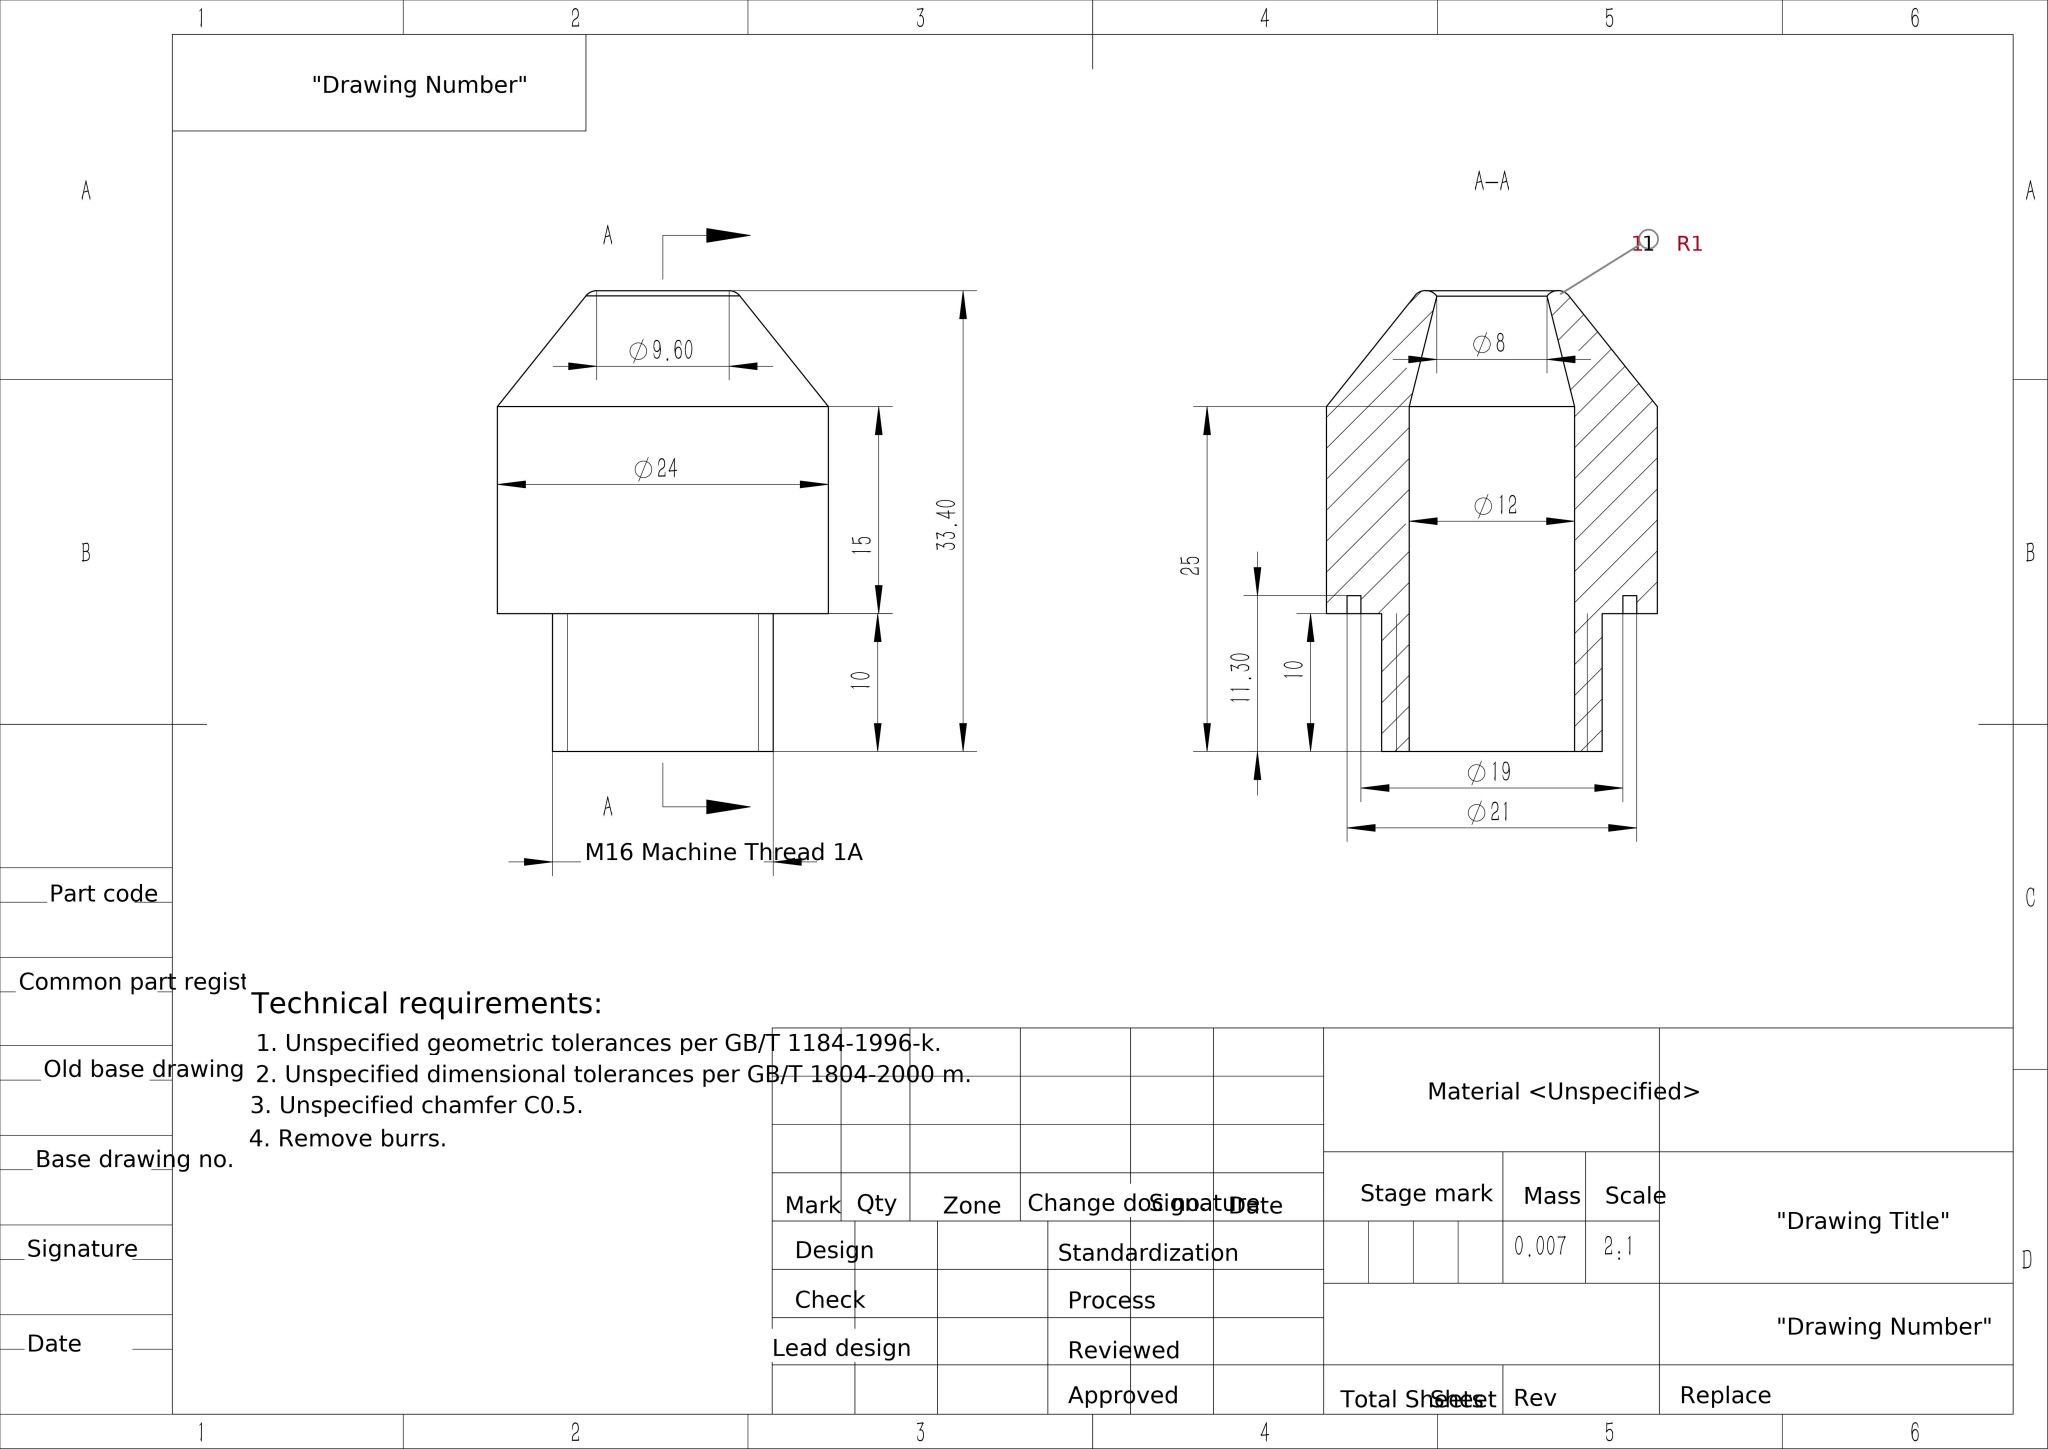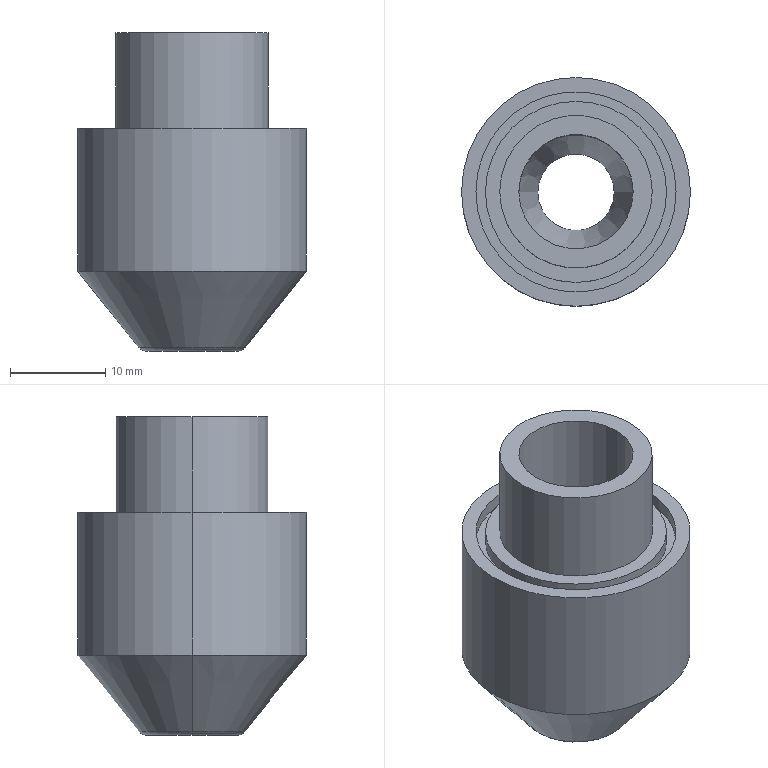Part | SolidWorks | mm | 1 solid | 20 faces | box 24 x 24 x 33.4 mm | volume 7296 mm3 | cylinder 10 | cone 4 | plane 4 | torus 2 | commonest cylinder face diameters 24 x2 12 x2 16 x2 21 x2 19 x2
STEP:
#1=CARTESIAN_POINT('',(5.581,0.,-8.024));
#2=VERTEX_POINT('',#1);
#3=CARTESIAN_POINT('',(-5.581,0.,-8.024));
#4=VERTEX_POINT('',#3);
#5=CARTESIAN_POINT('',(0.,0.,-8.024));
#6=DIRECTION('',(0.,0.,1.));
#7=DIRECTION('',(1.,0.,0.));
#8=AXIS2_PLACEMENT_3D('',#5,#6,#7);
#9=CIRCLE('',#8,5.581);
#10=EDGE_CURVE('',#2,#4,#9,.T.);
#11=ORIENTED_EDGE('',*,*,#10,.T.);
#12=CARTESIAN_POINT('',(-12.,0.,0.));
#13=VERTEX_POINT('',#12);
#14=CARTESIAN_POINT('',(-4.,0.,-10.));
#15=DIRECTION('',(-0.6247,0.,0.7809));
#16=VECTOR('',#15,1000.);
#17=LINE('',#14,#16);
#18=EDGE_CURVE('',#4,#13,#17,.T.);
#19=ORIENTED_EDGE('',*,*,#18,.T.);
#20=CARTESIAN_POINT('',(12.,0.,0.));
#21=VERTEX_POINT('',#20);
#22=CARTESIAN_POINT('',(0.,0.,0.));
#23=DIRECTION('',(0.,0.,1.));
#24=DIRECTION('',(1.,0.,0.));
#25=AXIS2_PLACEMENT_3D('',#22,#23,#24);
#26=CIRCLE('',#25,12.);
#27=EDGE_CURVE('',#21,#13,#26,.T.);
#28=ORIENTED_EDGE('',*,*,#27,.F.);
#29=CARTESIAN_POINT('',(4.,0.,-10.));
#30=DIRECTION('',(0.6247,0.,0.7809));
#31=VECTOR('',#30,1000.);
#32=LINE('',#29,#31);
#33=EDGE_CURVE('',#2,#21,#32,.T.);
#34=ORIENTED_EDGE('',*,*,#33,.F.);
#35=EDGE_LOOP('',(#11,#19,#28,#34));
#36=FACE_OUTER_BOUND('',#35,.T.);
#37=CARTESIAN_POINT('',(0.,0.,-10.));
#38=DIRECTION('',(0.,0.,1.));
#39=DIRECTION('',(1.,0.,0.));
#40=AXIS2_PLACEMENT_3D('',#37,#38,#39);
#41=CONICAL_SURFACE('',#40,4.,0.6747);
#42=ADVANCED_FACE('',(#36),#41,.T.);
#43=CARTESIAN_POINT('',(4.,0.,-8.));
#44=VERTEX_POINT('',#43);
#45=CARTESIAN_POINT('',(-4.,0.,-8.));
#46=VERTEX_POINT('',#45);
#47=CARTESIAN_POINT('',(0.,0.,-8.));
#48=DIRECTION('',(0.,0.,-1.));
#49=DIRECTION('',(1.,0.,0.));
#50=AXIS2_PLACEMENT_3D('',#47,#48,#49);
#51=CIRCLE('',#50,4.);
#52=EDGE_CURVE('',#44,#46,#51,.T.);
#53=ORIENTED_EDGE('',*,*,#52,.T.);
#54=CARTESIAN_POINT('',(-6.,0.,0.));
#55=VERTEX_POINT('',#54);
#56=CARTESIAN_POINT('',(-4.,0.,-8.));
#57=DIRECTION('',(-0.2425,0.,0.9701));
#58=VECTOR('',#57,1000.);
#59=LINE('',#56,#58);
#60=EDGE_CURVE('',#46,#55,#59,.T.);
#61=ORIENTED_EDGE('',*,*,#60,.T.);
#62=CARTESIAN_POINT('',(6.,0.,0.));
#63=VERTEX_POINT('',#62);
#64=CARTESIAN_POINT('',(0.,0.,0.));
#65=DIRECTION('',(0.,0.,-1.));
#66=DIRECTION('',(1.,0.,0.));
#67=AXIS2_PLACEMENT_3D('',#64,#65,#66);
#68=CIRCLE('',#67,6.);
#69=EDGE_CURVE('',#63,#55,#68,.T.);
#70=ORIENTED_EDGE('',*,*,#69,.F.);
#71=CARTESIAN_POINT('',(4.,0.,-8.));
#72=DIRECTION('',(0.2425,0.,0.9701));
#73=VECTOR('',#72,1000.);
#74=LINE('',#71,#73);
#75=EDGE_CURVE('',#44,#63,#74,.T.);
#76=ORIENTED_EDGE('',*,*,#75,.F.);
#77=EDGE_LOOP('',(#53,#61,#70,#76));
#78=FACE_OUTER_BOUND('',#77,.T.);
#79=CARTESIAN_POINT('',(0.,0.,-8.));
#80=DIRECTION('',(0.,0.,1.));
#81=DIRECTION('',(1.,0.,0.));
#82=AXIS2_PLACEMENT_3D('',#79,#80,#81);
#83=CONICAL_SURFACE('',#82,4.,0.245);
#84=ADVANCED_FACE('',(#78),#83,.F.);
#85=CARTESIAN_POINT('',(12.,0.,15.));
#86=VERTEX_POINT('',#85);
#87=CARTESIAN_POINT('',(-12.,0.,15.));
#88=VERTEX_POINT('',#87);
#89=CARTESIAN_POINT('',(0.,0.,15.));
#90=DIRECTION('',(0.,0.,1.));
#91=DIRECTION('',(1.,0.,0.));
#92=AXIS2_PLACEMENT_3D('',#89,#90,#91);
#93=CIRCLE('',#92,12.);
#94=EDGE_CURVE('',#86,#88,#93,.T.);
#95=ORIENTED_EDGE('',*,*,#94,.F.);
#96=CARTESIAN_POINT('',(12.,0.,15.));
#97=DIRECTION('',(0.,0.,-1.));
#98=VECTOR('',#97,1000.);
#99=LINE('',#96,#98);
#100=EDGE_CURVE('',#86,#21,#99,.T.);
#101=ORIENTED_EDGE('',*,*,#100,.T.);
#102=ORIENTED_EDGE('',*,*,#27,.T.);
#103=CARTESIAN_POINT('',(-12.,0.,15.));
#104=DIRECTION('',(0.,0.,-1.));
#105=VECTOR('',#104,1000.);
#106=LINE('',#103,#105);
#107=EDGE_CURVE('',#88,#13,#106,.T.);
#108=ORIENTED_EDGE('',*,*,#107,.F.);
#109=EDGE_LOOP('',(#95,#101,#102,#108));
#110=FACE_OUTER_BOUND('',#109,.T.);
#111=CARTESIAN_POINT('',(0.,0.,15.));
#112=DIRECTION('',(0.,0.,-1.));
#113=DIRECTION('',(-1.,0.,0.));
#114=AXIS2_PLACEMENT_3D('',#111,#112,#113);
#115=CYLINDRICAL_SURFACE('',#114,12.);
#116=ADVANCED_FACE('',(#110),#115,.T.);
#117=CARTESIAN_POINT('',(-6.,0.,25.));
#118=VERTEX_POINT('',#117);
#119=CARTESIAN_POINT('',(6.,0.,25.));
#120=VERTEX_POINT('',#119);
#121=CARTESIAN_POINT('',(0.,0.,25.));
#122=DIRECTION('',(0.,0.,1.));
#123=DIRECTION('',(1.,0.,0.));
#124=AXIS2_PLACEMENT_3D('',#121,#122,#123);
#125=CIRCLE('',#124,6.);
#126=EDGE_CURVE('',#118,#120,#125,.T.);
#127=ORIENTED_EDGE('',*,*,#126,.T.);
#128=CARTESIAN_POINT('',(6.,0.,15.));
#129=DIRECTION('',(0.,0.,-1.));
#130=VECTOR('',#129,1000.);
#131=LINE('',#128,#130);
#132=EDGE_CURVE('',#120,#63,#131,.T.);
#133=ORIENTED_EDGE('',*,*,#132,.T.);
#134=ORIENTED_EDGE('',*,*,#69,.T.);
#135=CARTESIAN_POINT('',(-6.,0.,15.));
#136=DIRECTION('',(0.,0.,-1.));
#137=VECTOR('',#136,1000.);
#138=LINE('',#135,#137);
#139=EDGE_CURVE('',#118,#55,#138,.T.);
#140=ORIENTED_EDGE('',*,*,#139,.F.);
#141=EDGE_LOOP('',(#127,#133,#134,#140));
#142=FACE_OUTER_BOUND('',#141,.T.);
#143=CARTESIAN_POINT('',(0.,0.,15.));
#144=DIRECTION('',(0.,0.,-1.));
#145=DIRECTION('',(-1.,0.,0.));
#146=AXIS2_PLACEMENT_3D('',#143,#144,#145);
#147=CYLINDRICAL_SURFACE('',#146,6.);
#148=ADVANCED_FACE('',(#142),#147,.F.);
#149=CARTESIAN_POINT('',(8.,0.,25.));
#150=VERTEX_POINT('',#149);
#151=CARTESIAN_POINT('',(-8.,0.,25.));
#152=VERTEX_POINT('',#151);
#153=CARTESIAN_POINT('',(0.,0.,25.));
#154=DIRECTION('',(0.,0.,1.));
#155=DIRECTION('',(1.,0.,0.));
#156=AXIS2_PLACEMENT_3D('',#153,#154,#155);
#157=CIRCLE('',#156,8.);
#158=EDGE_CURVE('',#150,#152,#157,.T.);
#159=ORIENTED_EDGE('',*,*,#158,.F.);
#160=CARTESIAN_POINT('',(8.,0.,15.));
#161=VERTEX_POINT('',#160);
#162=CARTESIAN_POINT('',(8.,0.,25.));
#163=DIRECTION('',(0.,0.,-1.));
#164=VECTOR('',#163,1000.);
#165=LINE('',#162,#164);
#166=EDGE_CURVE('',#150,#161,#165,.T.);
#167=ORIENTED_EDGE('',*,*,#166,.T.);
#168=CARTESIAN_POINT('',(-8.,0.,15.));
#169=VERTEX_POINT('',#168);
#170=CARTESIAN_POINT('',(0.,0.,15.));
#171=DIRECTION('',(0.,0.,1.));
#172=DIRECTION('',(1.,0.,0.));
#173=AXIS2_PLACEMENT_3D('',#170,#171,#172);
#174=CIRCLE('',#173,8.);
#175=EDGE_CURVE('',#161,#169,#174,.T.);
#176=ORIENTED_EDGE('',*,*,#175,.T.);
#177=CARTESIAN_POINT('',(-8.,0.,25.));
#178=DIRECTION('',(0.,0.,-1.));
#179=VECTOR('',#178,1000.);
#180=LINE('',#177,#179);
#181=EDGE_CURVE('',#152,#169,#180,.T.);
#182=ORIENTED_EDGE('',*,*,#181,.F.);
#183=EDGE_LOOP('',(#159,#167,#176,#182));
#184=FACE_OUTER_BOUND('',#183,.T.);
#185=CARTESIAN_POINT('',(0.,0.,25.));
#186=DIRECTION('',(0.,0.,-1.));
#187=DIRECTION('',(-1.,0.,0.));
#188=AXIS2_PLACEMENT_3D('',#185,#186,#187);
#189=CYLINDRICAL_SURFACE('',#188,8.);
#190=ADVANCED_FACE('',(#184),#189,.T.);
#191=CARTESIAN_POINT('',(10.5,0.,13.7));
#192=VERTEX_POINT('',#191);
#193=CARTESIAN_POINT('',(-10.5,0.,13.7));
#194=VERTEX_POINT('',#193);
#195=CARTESIAN_POINT('',(0.,0.,13.7));
#196=DIRECTION('',(0.,0.,-1.));
#197=DIRECTION('',(1.,0.,0.));
#198=AXIS2_PLACEMENT_3D('',#195,#196,#197);
#199=CIRCLE('',#198,10.5);
#200=EDGE_CURVE('',#192,#194,#199,.T.);
#201=ORIENTED_EDGE('',*,*,#200,.T.);
#202=CARTESIAN_POINT('',(-10.5,0.,15.));
#203=VERTEX_POINT('',#202);
#204=CARTESIAN_POINT('',(-10.5,0.,13.7));
#205=DIRECTION('',(0.,0.,1.));
#206=VECTOR('',#205,1000.);
#207=LINE('',#204,#206);
#208=EDGE_CURVE('',#194,#203,#207,.T.);
#209=ORIENTED_EDGE('',*,*,#208,.T.);
#210=CARTESIAN_POINT('',(10.5,0.,15.));
#211=VERTEX_POINT('',#210);
#212=CARTESIAN_POINT('',(0.,0.,15.));
#213=DIRECTION('',(0.,0.,1.));
#214=DIRECTION('',(1.,0.,0.));
#215=AXIS2_PLACEMENT_3D('',#212,#213,#214);
#216=CIRCLE('',#215,10.5);
#217=EDGE_CURVE('',#203,#211,#216,.T.);
#218=ORIENTED_EDGE('',*,*,#217,.T.);
#219=CARTESIAN_POINT('',(10.5,0.,13.7));
#220=DIRECTION('',(0.,0.,1.));
#221=VECTOR('',#220,1000.);
#222=LINE('',#219,#221);
#223=EDGE_CURVE('',#192,#211,#222,.T.);
#224=ORIENTED_EDGE('',*,*,#223,.F.);
#225=EDGE_LOOP('',(#201,#209,#218,#224));
#226=FACE_OUTER_BOUND('',#225,.T.);
#227=CARTESIAN_POINT('',(0.,0.,13.7));
#228=DIRECTION('',(0.,0.,1.));
#229=DIRECTION('',(1.,0.,0.));
#230=AXIS2_PLACEMENT_3D('',#227,#228,#229);
#231=CYLINDRICAL_SURFACE('',#230,10.5);
#232=ADVANCED_FACE('',(#226),#231,.F.);
#233=CARTESIAN_POINT('',(-9.5,0.,13.7));
#234=VERTEX_POINT('',#233);
#235=CARTESIAN_POINT('',(9.5,0.,13.7));
#236=VERTEX_POINT('',#235);
#237=CARTESIAN_POINT('',(0.,0.,13.7));
#238=DIRECTION('',(0.,0.,-1.));
#239=DIRECTION('',(1.,0.,0.));
#240=AXIS2_PLACEMENT_3D('',#237,#238,#239);
#241=CIRCLE('',#240,9.5);
#242=EDGE_CURVE('',#234,#236,#241,.T.);
#243=ORIENTED_EDGE('',*,*,#242,.F.);
#244=CARTESIAN_POINT('',(-9.5,0.,15.));
#245=VERTEX_POINT('',#244);
#246=CARTESIAN_POINT('',(-9.5,0.,13.7));
#247=DIRECTION('',(0.,0.,1.));
#248=VECTOR('',#247,1000.);
#249=LINE('',#246,#248);
#250=EDGE_CURVE('',#234,#245,#249,.T.);
#251=ORIENTED_EDGE('',*,*,#250,.T.);
#252=CARTESIAN_POINT('',(9.5,0.,15.));
#253=VERTEX_POINT('',#252);
#254=CARTESIAN_POINT('',(0.,0.,15.));
#255=DIRECTION('',(0.,0.,1.));
#256=DIRECTION('',(1.,0.,0.));
#257=AXIS2_PLACEMENT_3D('',#254,#255,#256);
#258=CIRCLE('',#257,9.5);
#259=EDGE_CURVE('',#253,#245,#258,.T.);
#260=ORIENTED_EDGE('',*,*,#259,.F.);
#261=CARTESIAN_POINT('',(9.5,0.,13.7));
#262=DIRECTION('',(0.,0.,1.));
#263=VECTOR('',#262,1000.);
#264=LINE('',#261,#263);
#265=EDGE_CURVE('',#236,#253,#264,.T.);
#266=ORIENTED_EDGE('',*,*,#265,.F.);
#267=EDGE_LOOP('',(#243,#251,#260,#266));
#268=FACE_OUTER_BOUND('',#267,.T.);
#269=CARTESIAN_POINT('',(0.,0.,13.7));
#270=DIRECTION('',(0.,0.,1.));
#271=DIRECTION('',(1.,0.,0.));
#272=AXIS2_PLACEMENT_3D('',#269,#270,#271);
#273=CYLINDRICAL_SURFACE('',#272,9.5);
#274=ADVANCED_FACE('',(#268),#273,.T.);
#275=ORIENTED_EDGE('',*,*,#10,.F.);
#276=CARTESIAN_POINT('',(4.8,0.,-7.4));
#277=DIRECTION('',(-0.,1.,0.));
#278=DIRECTION('',(-1.,-0.,0.));
#279=AXIS2_PLACEMENT_3D('',#276,#277,#278);
#280=CIRCLE('',#279,1.);
#281=EDGE_CURVE('',#2,#44,#280,.T.);
#282=ORIENTED_EDGE('',*,*,#281,.T.);
#283=CARTESIAN_POINT('',(0.,0.,-8.));
#284=DIRECTION('',(0.,0.,-1.));
#285=DIRECTION('',(1.,0.,0.));
#286=AXIS2_PLACEMENT_3D('',#283,#284,#285);
#287=CIRCLE('',#286,4.);
#288=EDGE_CURVE('',#46,#44,#287,.T.);
#289=ORIENTED_EDGE('',*,*,#288,.F.);
#290=CARTESIAN_POINT('',(-4.8,0.,-7.4));
#291=DIRECTION('',(0.,-1.,0.));
#292=DIRECTION('',(0.,0.,-1.));
#293=AXIS2_PLACEMENT_3D('',#290,#291,#292);
#294=CIRCLE('',#293,1.);
#295=EDGE_CURVE('',#4,#46,#294,.T.);
#296=ORIENTED_EDGE('',*,*,#295,.F.);
#297=EDGE_LOOP('',(#275,#282,#289,#296));
#298=FACE_OUTER_BOUND('',#297,.T.);
#299=CARTESIAN_POINT('',(0.,0.,-7.4));
#300=DIRECTION('',(0.,0.,-1.));
#301=DIRECTION('',(-1.,0.,0.));
#302=AXIS2_PLACEMENT_3D('',#299,#300,#301);
#303=TOROIDAL_SURFACE('',#302,4.8,1.);
#304=ADVANCED_FACE('',(#298),#303,.T.);
#305=ORIENTED_EDGE('',*,*,#281,.F.);
#306=CARTESIAN_POINT('',(0.,0.,-8.024));
#307=DIRECTION('',(0.,0.,1.));
#308=DIRECTION('',(1.,0.,0.));
#309=AXIS2_PLACEMENT_3D('',#306,#307,#308);
#310=CIRCLE('',#309,5.581);
#311=EDGE_CURVE('',#4,#2,#310,.T.);
#312=ORIENTED_EDGE('',*,*,#311,.F.);
#313=ORIENTED_EDGE('',*,*,#295,.T.);
#314=ORIENTED_EDGE('',*,*,#52,.F.);
#315=EDGE_LOOP('',(#305,#312,#313,#314));
#316=FACE_OUTER_BOUND('',#315,.T.);
#317=CARTESIAN_POINT('',(0.,0.,-7.4));
#318=DIRECTION('',(0.,0.,-1.));
#319=DIRECTION('',(-1.,0.,0.));
#320=AXIS2_PLACEMENT_3D('',#317,#318,#319);
#321=TOROIDAL_SURFACE('',#320,4.8,1.);
#322=ADVANCED_FACE('',(#316),#321,.T.);
#323=CARTESIAN_POINT('',(0.,0.,13.7));
#324=DIRECTION('',(0.,0.,-1.));
#325=DIRECTION('',(1.,0.,0.));
#326=AXIS2_PLACEMENT_3D('',#323,#324,#325);
#327=CIRCLE('',#326,9.5);
#328=EDGE_CURVE('',#236,#234,#327,.T.);
#329=ORIENTED_EDGE('',*,*,#328,.T.);
#330=ORIENTED_EDGE('',*,*,#242,.T.);
#331=EDGE_LOOP('',(#329,#330));
#332=FACE_BOUND('',#331,.T.);
#333=ORIENTED_EDGE('',*,*,#200,.F.);
#334=CARTESIAN_POINT('',(0.,0.,13.7));
#335=DIRECTION('',(0.,0.,-1.));
#336=DIRECTION('',(1.,0.,0.));
#337=AXIS2_PLACEMENT_3D('',#334,#335,#336);
#338=CIRCLE('',#337,10.5);
#339=EDGE_CURVE('',#194,#192,#338,.T.);
#340=ORIENTED_EDGE('',*,*,#339,.F.);
#341=EDGE_LOOP('',(#333,#340));
#342=FACE_OUTER_BOUND('',#341,.T.);
#343=CARTESIAN_POINT('',(0.,0.,13.7));
#344=DIRECTION('',(0.,0.,1.));
#345=DIRECTION('',(1.,0.,0.));
#346=AXIS2_PLACEMENT_3D('',#343,#344,#345);
#347=PLANE('',#346);
#348=ADVANCED_FACE('',(#332,#342),#347,.T.);
#349=ORIENTED_EDGE('',*,*,#250,.F.);
#350=ORIENTED_EDGE('',*,*,#328,.F.);
#351=ORIENTED_EDGE('',*,*,#265,.T.);
#352=CARTESIAN_POINT('',(0.,0.,15.));
#353=DIRECTION('',(0.,0.,1.));
#354=DIRECTION('',(1.,0.,0.));
#355=AXIS2_PLACEMENT_3D('',#352,#353,#354);
#356=CIRCLE('',#355,9.5);
#357=EDGE_CURVE('',#245,#253,#356,.T.);
#358=ORIENTED_EDGE('',*,*,#357,.F.);
#359=EDGE_LOOP('',(#349,#350,#351,#358));
#360=FACE_OUTER_BOUND('',#359,.T.);
#361=CARTESIAN_POINT('',(0.,0.,13.7));
#362=DIRECTION('',(0.,0.,1.));
#363=DIRECTION('',(1.,0.,0.));
#364=AXIS2_PLACEMENT_3D('',#361,#362,#363);
#365=CYLINDRICAL_SURFACE('',#364,9.5);
#366=ADVANCED_FACE('',(#360),#365,.T.);
#367=ORIENTED_EDGE('',*,*,#208,.F.);
#368=ORIENTED_EDGE('',*,*,#339,.T.);
#369=ORIENTED_EDGE('',*,*,#223,.T.);
#370=CARTESIAN_POINT('',(0.,0.,15.));
#371=DIRECTION('',(0.,0.,1.));
#372=DIRECTION('',(1.,0.,0.));
#373=AXIS2_PLACEMENT_3D('',#370,#371,#372);
#374=CIRCLE('',#373,10.5);
#375=EDGE_CURVE('',#211,#203,#374,.T.);
#376=ORIENTED_EDGE('',*,*,#375,.T.);
#377=EDGE_LOOP('',(#367,#368,#369,#376));
#378=FACE_OUTER_BOUND('',#377,.T.);
#379=CARTESIAN_POINT('',(0.,0.,13.7));
#380=DIRECTION('',(0.,0.,1.));
#381=DIRECTION('',(1.,0.,0.));
#382=AXIS2_PLACEMENT_3D('',#379,#380,#381);
#383=CYLINDRICAL_SURFACE('',#382,10.5);
#384=ADVANCED_FACE('',(#378),#383,.F.);
#385=ORIENTED_EDGE('',*,*,#126,.F.);
#386=CARTESIAN_POINT('',(0.,0.,25.));
#387=DIRECTION('',(0.,0.,1.));
#388=DIRECTION('',(1.,0.,0.));
#389=AXIS2_PLACEMENT_3D('',#386,#387,#388);
#390=CIRCLE('',#389,6.);
#391=EDGE_CURVE('',#120,#118,#390,.T.);
#392=ORIENTED_EDGE('',*,*,#391,.F.);
#393=EDGE_LOOP('',(#385,#392));
#394=FACE_BOUND('',#393,.T.);
#395=CARTESIAN_POINT('',(0.,0.,25.));
#396=DIRECTION('',(0.,0.,1.));
#397=DIRECTION('',(1.,0.,0.));
#398=AXIS2_PLACEMENT_3D('',#395,#396,#397);
#399=CIRCLE('',#398,8.);
#400=EDGE_CURVE('',#152,#150,#399,.T.);
#401=ORIENTED_EDGE('',*,*,#400,.T.);
#402=ORIENTED_EDGE('',*,*,#158,.T.);
#403=EDGE_LOOP('',(#401,#402));
#404=FACE_OUTER_BOUND('',#403,.T.);
#405=CARTESIAN_POINT('',(0.,0.,25.));
#406=DIRECTION('',(0.,0.,1.));
#407=DIRECTION('',(1.,0.,0.));
#408=AXIS2_PLACEMENT_3D('',#405,#406,#407);
#409=PLANE('',#408);
#410=ADVANCED_FACE('',(#394,#404),#409,.T.);
#411=ORIENTED_EDGE('',*,*,#166,.F.);
#412=ORIENTED_EDGE('',*,*,#400,.F.);
#413=ORIENTED_EDGE('',*,*,#181,.T.);
#414=CARTESIAN_POINT('',(0.,0.,15.));
#415=DIRECTION('',(0.,0.,1.));
#416=DIRECTION('',(1.,0.,0.));
#417=AXIS2_PLACEMENT_3D('',#414,#415,#416);
#418=CIRCLE('',#417,8.);
#419=EDGE_CURVE('',#169,#161,#418,.T.);
#420=ORIENTED_EDGE('',*,*,#419,.T.);
#421=EDGE_LOOP('',(#411,#412,#413,#420));
#422=FACE_OUTER_BOUND('',#421,.T.);
#423=CARTESIAN_POINT('',(0.,0.,25.));
#424=DIRECTION('',(0.,0.,-1.));
#425=DIRECTION('',(-1.,0.,0.));
#426=AXIS2_PLACEMENT_3D('',#423,#424,#425);
#427=CYLINDRICAL_SURFACE('',#426,8.);
#428=ADVANCED_FACE('',(#422),#427,.T.);
#429=CARTESIAN_POINT('',(0.,0.,15.));
#430=DIRECTION('',(0.,0.,1.));
#431=DIRECTION('',(1.,0.,0.));
#432=AXIS2_PLACEMENT_3D('',#429,#430,#431);
#433=CIRCLE('',#432,12.);
#434=EDGE_CURVE('',#88,#86,#433,.T.);
#435=ORIENTED_EDGE('',*,*,#434,.T.);
#436=ORIENTED_EDGE('',*,*,#94,.T.);
#437=EDGE_LOOP('',(#435,#436));
#438=FACE_OUTER_BOUND('',#437,.T.);
#439=ORIENTED_EDGE('',*,*,#375,.F.);
#440=ORIENTED_EDGE('',*,*,#217,.F.);
#441=EDGE_LOOP('',(#439,#440));
#442=FACE_BOUND('',#441,.T.);
#443=CARTESIAN_POINT('',(0.,0.,15.));
#444=DIRECTION('',(0.,0.,1.));
#445=DIRECTION('',(1.,0.,0.));
#446=AXIS2_PLACEMENT_3D('',#443,#444,#445);
#447=PLANE('',#446);
#448=ADVANCED_FACE('',(#438,#442),#447,.T.);
#449=ORIENTED_EDGE('',*,*,#132,.F.);
#450=ORIENTED_EDGE('',*,*,#391,.T.);
#451=ORIENTED_EDGE('',*,*,#139,.T.);
#452=CARTESIAN_POINT('',(0.,0.,0.));
#453=DIRECTION('',(0.,0.,-1.));
#454=DIRECTION('',(1.,0.,0.));
#455=AXIS2_PLACEMENT_3D('',#452,#453,#454);
#456=CIRCLE('',#455,6.);
#457=EDGE_CURVE('',#55,#63,#456,.T.);
#458=ORIENTED_EDGE('',*,*,#457,.T.);
#459=EDGE_LOOP('',(#449,#450,#451,#458));
#460=FACE_OUTER_BOUND('',#459,.T.);
#461=CARTESIAN_POINT('',(0.,0.,15.));
#462=DIRECTION('',(0.,0.,-1.));
#463=DIRECTION('',(-1.,0.,0.));
#464=AXIS2_PLACEMENT_3D('',#461,#462,#463);
#465=CYLINDRICAL_SURFACE('',#464,6.);
#466=ADVANCED_FACE('',(#460),#465,.F.);
#467=ORIENTED_EDGE('',*,*,#100,.F.);
#468=ORIENTED_EDGE('',*,*,#434,.F.);
#469=ORIENTED_EDGE('',*,*,#107,.T.);
#470=CARTESIAN_POINT('',(0.,0.,0.));
#471=DIRECTION('',(0.,0.,1.));
#472=DIRECTION('',(1.,0.,0.));
#473=AXIS2_PLACEMENT_3D('',#470,#471,#472);
#474=CIRCLE('',#473,12.);
#475=EDGE_CURVE('',#13,#21,#474,.T.);
#476=ORIENTED_EDGE('',*,*,#475,.T.);
#477=EDGE_LOOP('',(#467,#468,#469,#476));
#478=FACE_OUTER_BOUND('',#477,.T.);
#479=CARTESIAN_POINT('',(0.,0.,15.));
#480=DIRECTION('',(0.,0.,-1.));
#481=DIRECTION('',(-1.,0.,0.));
#482=AXIS2_PLACEMENT_3D('',#479,#480,#481);
#483=CYLINDRICAL_SURFACE('',#482,12.);
#484=ADVANCED_FACE('',(#478),#483,.T.);
#485=ORIENTED_EDGE('',*,*,#60,.F.);
#486=ORIENTED_EDGE('',*,*,#288,.T.);
#487=ORIENTED_EDGE('',*,*,#75,.T.);
#488=ORIENTED_EDGE('',*,*,#457,.F.);
#489=EDGE_LOOP('',(#485,#486,#487,#488));
#490=FACE_OUTER_BOUND('',#489,.T.);
#491=CARTESIAN_POINT('',(0.,0.,-8.));
#492=DIRECTION('',(0.,0.,1.));
#493=DIRECTION('',(1.,0.,0.));
#494=AXIS2_PLACEMENT_3D('',#491,#492,#493);
#495=CONICAL_SURFACE('',#494,4.,0.245);
#496=ADVANCED_FACE('',(#490),#495,.F.);
#497=ORIENTED_EDGE('',*,*,#18,.F.);
#498=ORIENTED_EDGE('',*,*,#311,.T.);
#499=ORIENTED_EDGE('',*,*,#33,.T.);
#500=ORIENTED_EDGE('',*,*,#475,.F.);
#501=EDGE_LOOP('',(#497,#498,#499,#500));
#502=FACE_OUTER_BOUND('',#501,.T.);
#503=CARTESIAN_POINT('',(0.,0.,-10.));
#504=DIRECTION('',(0.,0.,1.));
#505=DIRECTION('',(1.,0.,0.));
#506=AXIS2_PLACEMENT_3D('',#503,#504,#505);
#507=CONICAL_SURFACE('',#506,4.,0.6747);
#508=ADVANCED_FACE('',(#502),#507,.T.);
#509=ORIENTED_EDGE('',*,*,#259,.T.);
#510=ORIENTED_EDGE('',*,*,#357,.T.);
#511=EDGE_LOOP('',(#509,#510));
#512=FACE_OUTER_BOUND('',#511,.T.);
#513=ORIENTED_EDGE('',*,*,#419,.F.);
#514=ORIENTED_EDGE('',*,*,#175,.F.);
#515=EDGE_LOOP('',(#513,#514));
#516=FACE_BOUND('',#515,.T.);
#517=CARTESIAN_POINT('',(0.,0.,15.));
#518=DIRECTION('',(0.,0.,1.));
#519=DIRECTION('',(1.,0.,0.));
#520=AXIS2_PLACEMENT_3D('',#517,#518,#519);
#521=PLANE('',#520);
#522=ADVANCED_FACE('',(#512,#516),#521,.T.);
#523=CLOSED_SHELL('',(#42,#84,#116,#148,#190,#232,#274,#304,#322,#348,#366,#384,#410,#428,#448,#466,#484,#496,#508,#522));
#524=MANIFOLD_SOLID_BREP('',#523);
#525=CARTESIAN_POINT('',(0.,0.,0.));
#526=DIRECTION('',(0.,0.,1.));
#527=DIRECTION('',(1.,0.,0.));
#528=AXIS2_PLACEMENT_3D('',#525,#526,#527);
#529=(LENGTH_UNIT()NAMED_UNIT(*)SI_UNIT(.MILLI.,.METRE.));
#530=UNCERTAINTY_MEASURE_WITH_UNIT(LENGTH_MEASURE(0.00001),#529,'','');
#531=(NAMED_UNIT(*)PLANE_ANGLE_UNIT()SI_UNIT($,.RADIAN.));
#532=(NAMED_UNIT(*)SI_UNIT($,.STERADIAN.)SOLID_ANGLE_UNIT());
#533=(GEOMETRIC_REPRESENTATION_CONTEXT(3)GLOBAL_UNCERTAINTY_ASSIGNED_CONTEXT((#530))GLOBAL_UNIT_ASSIGNED_CONTEXT((#529,#531,#532))REPRESENTATION_CONTEXT('',''));
#534=ADVANCED_BREP_SHAPE_REPRESENTATION('',(#524,#528),#533);